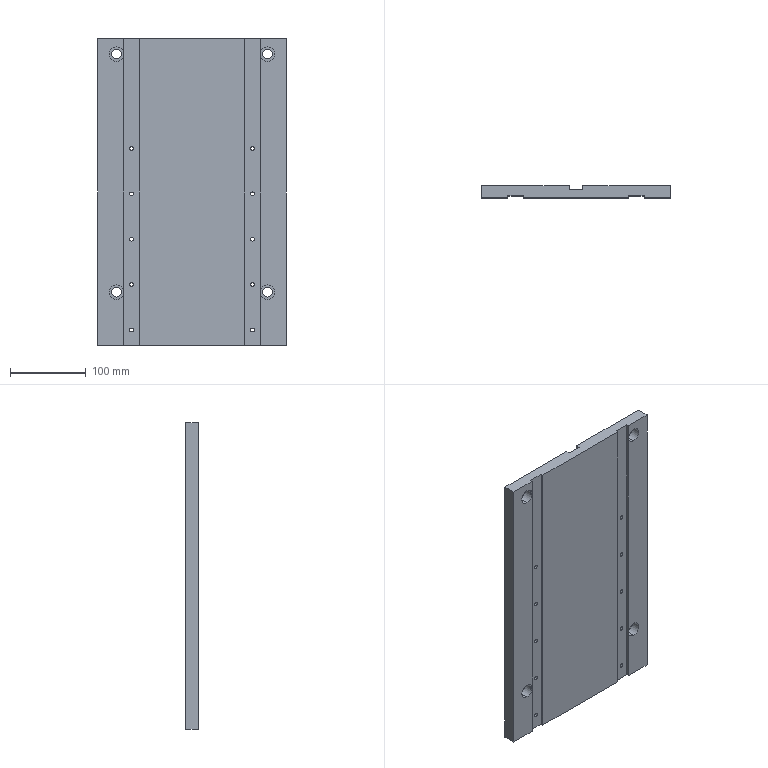Component | SolidWorks | NewTypeCurveBenderReinforcementSlideRailBasePlate-DoubleWheel-1 | 1 solid | 58 faces | box 250 x 16 x 405 mm | volume 1516664 mm3 | cylinder 36 | plane 22 | commonest cylinder face diameters 5 x20 19 x8 13 x8
build123d program:
from build123d import *

# Parameters (mm, degrees)
SKETCH1_W                      = 250
SKETCH1_H                      = 405
BOSS_EXTRUDE1_DEPTH            = 16
F_13_0_13_DIAMETER_HOLE1_D     = 13
F_13_0_13_DIAMETER_HOLE1_DEPTH = 28.75
F_13_0_13_DIAMETER_HOLE1_TIP   = 3.906
M6_TAPPED_HOLE1_D              = 5
SKETCH6_W                      = 20
SKETCH6_H                      = 6
SKETCH6_W_2                    = 18
SKETCH6_H_2                    = 10
CUT_EXTRUDE1_DEPTH             = 425.153
SKETCH7_R                      = 9.5
CUT_EXTRUDE2_DEPTH             = 12


with BuildPart() as part:
    # Sketch1 → Boss-Extrude1 (new body)
    with BuildSketch(Plane(origin=(0, 0, 0), x_dir=(1, 0, 0), z_dir=(0, 1, 0))):
        Rectangle(SKETCH1_W, SKETCH1_H)
    extrude(amount=BOSS_EXTRUDE1_DEPTH)

    # 13.0 _13_ Diameter Hole1
    with Locations(Plane(origin=(0, 16, 0), x_dir=(1, 0, 0), z_dir=(0, 1, 0))):
        with Locations((-100, 182.5), (-100, -132.5), (100, -132.5), (100, 182.5)):
            Hole(F_13_0_13_DIAMETER_HOLE1_D / 2, depth=F_13_0_13_DIAMETER_HOLE1_DEPTH)
            with Locations((0, 0, -(F_13_0_13_DIAMETER_HOLE1_DEPTH + F_13_0_13_DIAMETER_HOLE1_TIP / 2))):  # 118° drill point
                Cone(0, F_13_0_13_DIAMETER_HOLE1_D / 2, F_13_0_13_DIAMETER_HOLE1_TIP, mode=Mode.SUBTRACT)

    # M6 Tapped Hole1 (through all)
    with Locations(Plane(origin=(0, 16, 0), x_dir=(1, 0, 0), z_dir=(0, 1, 0))):
        with Locations((-80, -182.5), (-80, -122.5), (-80, -62.5), (-80, -2.5), (80, -2.5), (80, -62.5), (80, -122.5), (80, -182.5), (-80, 57.5), (80, 57.5)):
            Hole(M6_TAPPED_HOLE1_D / 2)

    # Sketch6 → Cut-Extrude1 (cut, through all)
    with BuildSketch(Plane.XY.offset(202.5)):
        with Locations((-80, 16)):
            Rectangle(SKETCH6_W, SKETCH6_H)
        with Locations((80, 16)):
            Rectangle(SKETCH6_W, SKETCH6_H)
        Rectangle(SKETCH6_W_2, SKETCH6_H_2)
    extrude(amount=-CUT_EXTRUDE1_DEPTH, mode=Mode.SUBTRACT)

    # Sketch7 → Cut-Extrude2 (cut)
    with BuildSketch(Plane(origin=(0, 16, 0), x_dir=(1, 0, 0), z_dir=(0, 1, 0))):
        with Locations(Location((-100, 182.5, 0), (0, 0, 270))):
            Circle(SKETCH7_R)
        with Locations(Location((100, 182.5, 0), (0, 0, 270))):
            Circle(SKETCH7_R)
        with Locations(Location((100, -132.5, 0), (0, 0, 270))):
            Circle(SKETCH7_R)
        with Locations(Location((-100, -132.5, 0), (0, 0, 270))):
            Circle(SKETCH7_R)
    extrude(amount=-CUT_EXTRUDE2_DEPTH, mode=Mode.SUBTRACT)


solid = part.part

# Placed as in the assembly
solid = solid.moved(Location((0, 76, 70.61), (180, 0, 0)))